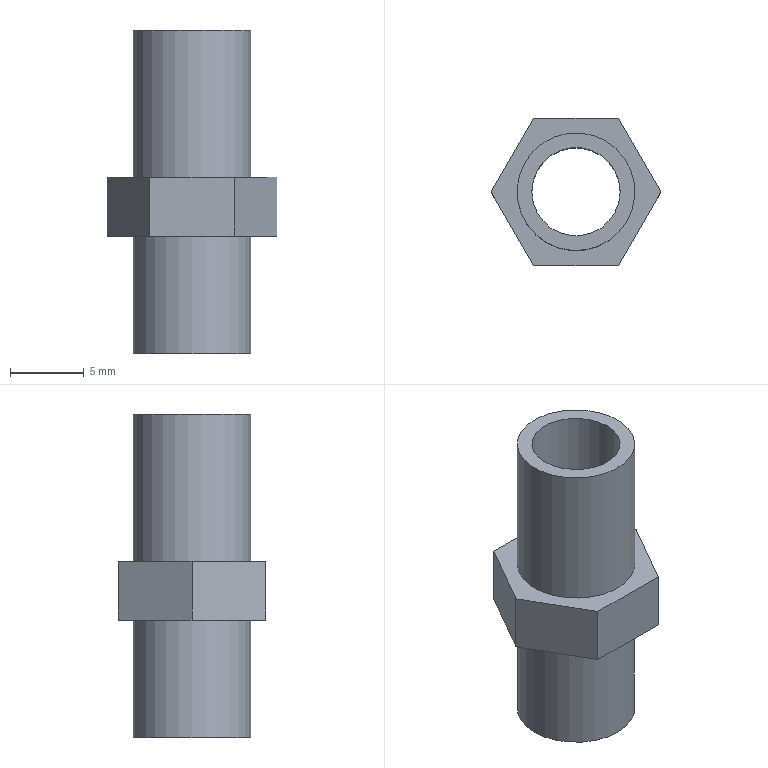Component | NX | PIPE_CAP_2_2 | 1 solid | 13 faces | box 11.55 x 10 x 22 mm | volume 629 mm3 | plane 10 | cylinder 3 | commonest cylinder face diameters 8 x2 6 x1
STEP:
#1=CARTESIAN_POINT('',(0.,0.,0.));
#2=DIRECTION('',(0.,0.,1.));
#3=DIRECTION('',(1.,0.,0.));
#4=AXIS2_PLACEMENT_3D('',#1,#2,#3);
#5=CARTESIAN_POINT('',(-114.5,-59.,24.5));
#6=VERTEX_POINT('',#5);
#7=CARTESIAN_POINT('',(-108.5,-59.,24.5));
#8=VERTEX_POINT('',#7);
#9=CARTESIAN_POINT('',(-111.5,-59.,24.5));
#10=DIRECTION('',(0.,0.,-1.));
#11=DIRECTION('',(-1.,0.,0.));
#12=AXIS2_PLACEMENT_3D('',#9,#10,#11);
#13=CIRCLE('',#12,3.);
#14=CARTESIAN_POINT('',(-111.5,-59.,24.5));
#15=DIRECTION('',(0.,0.,-1.));
#16=DIRECTION('',(-1.,0.,0.));
#17=AXIS2_PLACEMENT_3D('',#14,#15,#16);
#18=PLANE('',#17);
#19=CARTESIAN_POINT('',(0.,0.));
#20=DIRECTION('',(1.,0.));
#21=AXIS2_PLACEMENT_2D('',#19,#20);
#22=CIRCLE('',#21,3.);
#23=(GEOMETRIC_REPRESENTATION_CONTEXT(2)PARAMETRIC_REPRESENTATION_CONTEXT()REPRESENTATION_CONTEXT('',''));
#24=DEFINITIONAL_REPRESENTATION('',(#22),#23);
#25=PCURVE('',#18,#24);
#26=CARTESIAN_POINT('',(-111.5,-59.,-3.5));
#27=DIRECTION('',(0.,0.,1.));
#28=DIRECTION('',(1.,0.,0.));
#29=AXIS2_PLACEMENT_3D('',#26,#27,#28);
#30=CYLINDRICAL_SURFACE('',#29,3.);
#31=CARTESIAN_POINT('',(3.142,28.));
#32=DIRECTION('',(-1.,0.));
#33=VECTOR('',#32,1.);
#34=LINE('',#31,#33);
#35=(GEOMETRIC_REPRESENTATION_CONTEXT(2)PARAMETRIC_REPRESENTATION_CONTEXT()REPRESENTATION_CONTEXT('',''));
#36=DEFINITIONAL_REPRESENTATION('',(#34),#35);
#37=PCURVE('',#30,#36);
#38=SURFACE_CURVE('',#13,(#25,#37),.PCURVE_S1.);
#39=EDGE_CURVE('',#6,#8,#38,.T.);
#40=ORIENTED_EDGE('',*,*,#39,.F.);
#41=CARTESIAN_POINT('',(-111.5,-59.,24.5));
#42=DIRECTION('',(0.,0.,-1.));
#43=DIRECTION('',(-1.,0.,0.));
#44=AXIS2_PLACEMENT_3D('',#41,#42,#43);
#45=CIRCLE('',#44,3.);
#46=CARTESIAN_POINT('',(0.,0.));
#47=DIRECTION('',(1.,0.));
#48=AXIS2_PLACEMENT_2D('',#46,#47);
#49=CIRCLE('',#48,3.);
#50=(GEOMETRIC_REPRESENTATION_CONTEXT(2)PARAMETRIC_REPRESENTATION_CONTEXT()REPRESENTATION_CONTEXT('',''));
#51=DEFINITIONAL_REPRESENTATION('',(#49),#50);
#52=PCURVE('',#18,#51);
#53=CARTESIAN_POINT('',(9.425,28.));
#54=DIRECTION('',(-1.,0.));
#55=VECTOR('',#54,1.);
#56=LINE('',#53,#55);
#57=(GEOMETRIC_REPRESENTATION_CONTEXT(2)PARAMETRIC_REPRESENTATION_CONTEXT()REPRESENTATION_CONTEXT('',''));
#58=DEFINITIONAL_REPRESENTATION('',(#56),#57);
#59=PCURVE('',#30,#58);
#60=SURFACE_CURVE('',#45,(#52,#59),.PCURVE_S1.);
#61=EDGE_CURVE('',#8,#6,#60,.T.);
#62=ORIENTED_EDGE('',*,*,#61,.F.);
#63=EDGE_LOOP('',(#40,#62));
#64=FACE_BOUND('',#63,.T.);
#65=CARTESIAN_POINT('',(-107.5,-59.,24.5));
#66=VERTEX_POINT('',#65);
#67=CARTESIAN_POINT('',(-111.5,-59.,24.5));
#68=DIRECTION('',(0.,0.,1.));
#69=DIRECTION('',(1.,0.,0.));
#70=AXIS2_PLACEMENT_3D('',#67,#68,#69);
#71=CIRCLE('',#70,4.);
#72=CARTESIAN_POINT('',(-4.,0.));
#73=CARTESIAN_POINT('',(-4.,6.928));
#74=CARTESIAN_POINT('',(2.,3.464));
#75=CARTESIAN_POINT('',(8.,0.));
#76=CARTESIAN_POINT('',(2.,-3.464));
#77=CARTESIAN_POINT('',(-4.,-6.928));
#78=CARTESIAN_POINT('',(-4.,0.));
#79=(BOUNDED_CURVE()B_SPLINE_CURVE(2,(#72,#73,#74,#75,#76,#77,#78),.UNSPECIFIED.,.T.,.F.)B_SPLINE_CURVE_WITH_KNOTS((1,2,2,2,2,1),(-2.094,0.,2.094,4.189,6.283,8.378),.UNSPECIFIED.)CURVE()GEOMETRIC_REPRESENTATION_ITEM()RATIONAL_B_SPLINE_CURVE((1.,0.5,1.,0.5,1.,0.5,1.))REPRESENTATION_ITEM(''));
#80=(GEOMETRIC_REPRESENTATION_CONTEXT(2)PARAMETRIC_REPRESENTATION_CONTEXT()REPRESENTATION_CONTEXT('',''));
#81=DEFINITIONAL_REPRESENTATION('',(#79),#80);
#82=PCURVE('',#18,#81);
#83=CARTESIAN_POINT('',(-111.5,-59.,24.5));
#84=DIRECTION('',(0.,0.,1.));
#85=DIRECTION('',(1.,0.,0.));
#86=AXIS2_PLACEMENT_3D('',#83,#84,#85);
#87=CYLINDRICAL_SURFACE('',#86,4.);
#88=CARTESIAN_POINT('',(0.,0.));
#89=DIRECTION('',(1.,0.));
#90=VECTOR('',#89,1.);
#91=LINE('',#88,#90);
#92=(GEOMETRIC_REPRESENTATION_CONTEXT(2)PARAMETRIC_REPRESENTATION_CONTEXT()REPRESENTATION_CONTEXT('',''));
#93=DEFINITIONAL_REPRESENTATION('',(#91),#92);
#94=PCURVE('',#87,#93);
#95=SURFACE_CURVE('',#71,(#82,#94),.PCURVE_S1.);
#96=EDGE_CURVE('',#66,#66,#95,.T.);
#97=ORIENTED_EDGE('',*,*,#96,.F.);
#98=EDGE_LOOP('',(#97));
#99=FACE_BOUND('',#98,.T.);
#100=ADVANCED_FACE('',(#64,#99),#18,.T.);
#101=CARTESIAN_POINT('',(-107.5,-59.,32.5));
#102=VERTEX_POINT('',#101);
#103=CARTESIAN_POINT('',(-111.5,-59.,32.5));
#104=DIRECTION('',(0.,0.,-1.));
#105=DIRECTION('',(1.,0.,0.));
#106=AXIS2_PLACEMENT_3D('',#103,#104,#105);
#107=CIRCLE('',#106,4.);
#108=CARTESIAN_POINT('',(6.283,8.));
#109=DIRECTION('',(-1.,0.));
#110=VECTOR('',#109,1.);
#111=LINE('',#108,#110);
#112=(GEOMETRIC_REPRESENTATION_CONTEXT(2)PARAMETRIC_REPRESENTATION_CONTEXT()REPRESENTATION_CONTEXT('',''));
#113=DEFINITIONAL_REPRESENTATION('',(#111),#112);
#114=PCURVE('',#87,#113);
#115=CARTESIAN_POINT('',(-111.5,-59.,32.5));
#116=DIRECTION('',(0.,0.,-1.));
#117=DIRECTION('',(-1.,0.,0.));
#118=AXIS2_PLACEMENT_3D('',#115,#116,#117);
#119=PLANE('',#118);
#120=CARTESIAN_POINT('',(0.,0.));
#121=DIRECTION('',(-1.,0.));
#122=AXIS2_PLACEMENT_2D('',#120,#121);
#123=CIRCLE('',#122,4.);
#124=(GEOMETRIC_REPRESENTATION_CONTEXT(2)PARAMETRIC_REPRESENTATION_CONTEXT()REPRESENTATION_CONTEXT('',''));
#125=DEFINITIONAL_REPRESENTATION('',(#123),#124);
#126=PCURVE('',#119,#125);
#127=SURFACE_CURVE('',#107,(#114,#126),.PCURVE_S1.);
#128=EDGE_CURVE('',#102,#102,#127,.T.);
#129=ORIENTED_EDGE('',*,*,#128,.T.);
#130=CARTESIAN_POINT('',(-107.5,-59.,24.5));
#131=CARTESIAN_POINT('',(-107.5,-59.,32.5));
#132=B_SPLINE_CURVE_WITH_KNOTS('',1,(#130,#131),.UNSPECIFIED.,.F.,.F.,(2,2),(0.,8.),.PIECEWISE_BEZIER_KNOTS.);
#133=CARTESIAN_POINT('',(0.,0.));
#134=DIRECTION('',(0.,1.));
#135=VECTOR('',#134,1.);
#136=LINE('',#133,#135);
#137=(GEOMETRIC_REPRESENTATION_CONTEXT(2)PARAMETRIC_REPRESENTATION_CONTEXT()REPRESENTATION_CONTEXT('',''));
#138=DEFINITIONAL_REPRESENTATION('',(#136),#137);
#139=PCURVE('',#87,#138);
#140=CARTESIAN_POINT('',(6.283,0.));
#141=DIRECTION('',(0.,1.));
#142=VECTOR('',#141,1.);
#143=LINE('',#140,#142);
#144=(GEOMETRIC_REPRESENTATION_CONTEXT(2)PARAMETRIC_REPRESENTATION_CONTEXT()REPRESENTATION_CONTEXT('',''));
#145=DEFINITIONAL_REPRESENTATION('',(#143),#144);
#146=PCURVE('',#87,#145);
#147=SEAM_CURVE('',#132,(#139,#146),.PCURVE_S1.);
#148=EDGE_CURVE('',#66,#102,#147,.T.);
#149=ORIENTED_EDGE('',*,*,#148,.F.);
#150=ORIENTED_EDGE('',*,*,#96,.T.);
#151=ORIENTED_EDGE('',*,*,#148,.T.);
#152=EDGE_LOOP('',(#129,#149,#150,#151));
#153=FACE_BOUND('',#152,.T.);
#154=ADVANCED_FACE('',(#153),#87,.T.);
#155=CARTESIAN_POINT('',(-108.613,-54.,32.5));
#156=VERTEX_POINT('',#155);
#157=CARTESIAN_POINT('',(-105.726,-59.,32.5));
#158=VERTEX_POINT('',#157);
#159=CARTESIAN_POINT('',(-108.613,-54.,32.5));
#160=DIRECTION('',(0.5,-0.866,0.));
#161=VECTOR('',#160,1.);
#162=LINE('',#159,#161);
#163=CARTESIAN_POINT('',(-108.613,-54.,36.5));
#164=DIRECTION('',(0.866,0.5,0.));
#165=DIRECTION('',(-0.5,0.866,0.));
#166=AXIS2_PLACEMENT_3D('',#163,#164,#165);
#167=PLANE('',#166);
#168=CARTESIAN_POINT('',(0.,-4.));
#169=DIRECTION('',(-1.,0.));
#170=VECTOR('',#169,1.);
#171=LINE('',#168,#170);
#172=(GEOMETRIC_REPRESENTATION_CONTEXT(2)PARAMETRIC_REPRESENTATION_CONTEXT()REPRESENTATION_CONTEXT('',''));
#173=DEFINITIONAL_REPRESENTATION('',(#171),#172);
#174=PCURVE('',#167,#173);
#175=CARTESIAN_POINT('',(-2.887,5.));
#176=DIRECTION('',(-0.5,-0.866));
#177=VECTOR('',#176,1.);
#178=LINE('',#175,#177);
#179=(GEOMETRIC_REPRESENTATION_CONTEXT(2)PARAMETRIC_REPRESENTATION_CONTEXT()REPRESENTATION_CONTEXT('',''));
#180=DEFINITIONAL_REPRESENTATION('',(#178),#179);
#181=PCURVE('',#119,#180);
#182=SURFACE_CURVE('',#162,(#174,#181),.PCURVE_S1.);
#183=EDGE_CURVE('',#156,#158,#182,.T.);
#184=ORIENTED_EDGE('',*,*,#183,.F.);
#185=CARTESIAN_POINT('',(-108.613,-54.,36.5));
#186=VERTEX_POINT('',#185);
#187=CARTESIAN_POINT('',(-108.613,-54.,36.5));
#188=DIRECTION('',(0.,0.,-1.));
#189=VECTOR('',#188,1.);
#190=LINE('',#187,#189);
#191=CARTESIAN_POINT('',(0.,0.));
#192=DIRECTION('',(0.,-1.));
#193=VECTOR('',#192,1.);
#194=LINE('',#191,#193);
#195=(GEOMETRIC_REPRESENTATION_CONTEXT(2)PARAMETRIC_REPRESENTATION_CONTEXT()REPRESENTATION_CONTEXT('',''));
#196=DEFINITIONAL_REPRESENTATION('',(#194),#195);
#197=PCURVE('',#167,#196);
#198=CARTESIAN_POINT('',(-114.387,-54.,36.5));
#199=DIRECTION('',(0.,1.,0.));
#200=DIRECTION('',(0.,0.,1.));
#201=AXIS2_PLACEMENT_3D('',#198,#199,#200);
#202=PLANE('',#201);
#203=CARTESIAN_POINT('',(0.,5.774));
#204=DIRECTION('',(-1.,0.));
#205=VECTOR('',#204,1.);
#206=LINE('',#203,#205);
#207=(GEOMETRIC_REPRESENTATION_CONTEXT(2)PARAMETRIC_REPRESENTATION_CONTEXT()REPRESENTATION_CONTEXT('',''));
#208=DEFINITIONAL_REPRESENTATION('',(#206),#207);
#209=PCURVE('',#202,#208);
#210=SURFACE_CURVE('',#190,(#197,#209),.PCURVE_S1.);
#211=EDGE_CURVE('',#186,#156,#210,.T.);
#212=ORIENTED_EDGE('',*,*,#211,.F.);
#213=CARTESIAN_POINT('',(-105.726,-59.,36.5));
#214=VERTEX_POINT('',#213);
#215=CARTESIAN_POINT('',(-108.613,-54.,36.5));
#216=DIRECTION('',(0.5,-0.866,0.));
#217=VECTOR('',#216,1.);
#218=LINE('',#215,#217);
#219=CARTESIAN_POINT('',(0.,0.));
#220=DIRECTION('',(-1.,0.));
#221=VECTOR('',#220,1.);
#222=LINE('',#219,#221);
#223=(GEOMETRIC_REPRESENTATION_CONTEXT(2)PARAMETRIC_REPRESENTATION_CONTEXT()REPRESENTATION_CONTEXT('',''));
#224=DEFINITIONAL_REPRESENTATION('',(#222),#223);
#225=PCURVE('',#167,#224);
#226=CARTESIAN_POINT('',(-111.5,-59.,36.5));
#227=DIRECTION('',(0.,0.,-1.));
#228=DIRECTION('',(-1.,0.,0.));
#229=AXIS2_PLACEMENT_3D('',#226,#227,#228);
#230=PLANE('',#229);
#231=CARTESIAN_POINT('',(-2.887,5.));
#232=DIRECTION('',(-0.5,-0.866));
#233=VECTOR('',#232,1.);
#234=LINE('',#231,#233);
#235=(GEOMETRIC_REPRESENTATION_CONTEXT(2)PARAMETRIC_REPRESENTATION_CONTEXT()REPRESENTATION_CONTEXT('',''));
#236=DEFINITIONAL_REPRESENTATION('',(#234),#235);
#237=PCURVE('',#230,#236);
#238=SURFACE_CURVE('',#218,(#225,#237),.PCURVE_S1.);
#239=EDGE_CURVE('',#186,#214,#238,.T.);
#240=ORIENTED_EDGE('',*,*,#239,.T.);
#241=CARTESIAN_POINT('',(-105.726,-59.,36.5));
#242=DIRECTION('',(0.,0.,-1.));
#243=VECTOR('',#242,1.);
#244=LINE('',#241,#243);
#245=CARTESIAN_POINT('',(-5.774,0.));
#246=DIRECTION('',(0.,-1.));
#247=VECTOR('',#246,1.);
#248=LINE('',#245,#247);
#249=(GEOMETRIC_REPRESENTATION_CONTEXT(2)PARAMETRIC_REPRESENTATION_CONTEXT()REPRESENTATION_CONTEXT('',''));
#250=DEFINITIONAL_REPRESENTATION('',(#248),#249);
#251=PCURVE('',#167,#250);
#252=CARTESIAN_POINT('',(-105.726,-59.,36.5));
#253=DIRECTION('',(0.866,-0.5,0.));
#254=DIRECTION('',(0.5,0.866,0.));
#255=AXIS2_PLACEMENT_3D('',#252,#253,#254);
#256=PLANE('',#255);
#257=CARTESIAN_POINT('',(0.,0.));
#258=DIRECTION('',(0.,-1.));
#259=VECTOR('',#258,1.);
#260=LINE('',#257,#259);
#261=(GEOMETRIC_REPRESENTATION_CONTEXT(2)PARAMETRIC_REPRESENTATION_CONTEXT()REPRESENTATION_CONTEXT('',''));
#262=DEFINITIONAL_REPRESENTATION('',(#260),#261);
#263=PCURVE('',#256,#262);
#264=SURFACE_CURVE('',#244,(#251,#263),.PCURVE_S1.);
#265=EDGE_CURVE('',#214,#158,#264,.T.);
#266=ORIENTED_EDGE('',*,*,#265,.T.);
#267=EDGE_LOOP('',(#184,#212,#240,#266));
#268=FACE_BOUND('',#267,.T.);
#269=ADVANCED_FACE('',(#268),#167,.T.);
#270=CARTESIAN_POINT('',(-108.613,-64.,32.5));
#271=VERTEX_POINT('',#270);
#272=CARTESIAN_POINT('',(-105.726,-59.,32.5));
#273=DIRECTION('',(-0.5,-0.866,0.));
#274=VECTOR('',#273,1.);
#275=LINE('',#272,#274);
#276=CARTESIAN_POINT('',(0.,-4.));
#277=DIRECTION('',(-1.,0.));
#278=VECTOR('',#277,1.);
#279=LINE('',#276,#278);
#280=(GEOMETRIC_REPRESENTATION_CONTEXT(2)PARAMETRIC_REPRESENTATION_CONTEXT()REPRESENTATION_CONTEXT('',''));
#281=DEFINITIONAL_REPRESENTATION('',(#279),#280);
#282=PCURVE('',#256,#281);
#283=CARTESIAN_POINT('',(-5.774,0.));
#284=DIRECTION('',(0.5,-0.866));
#285=VECTOR('',#284,1.);
#286=LINE('',#283,#285);
#287=(GEOMETRIC_REPRESENTATION_CONTEXT(2)PARAMETRIC_REPRESENTATION_CONTEXT()REPRESENTATION_CONTEXT('',''));
#288=DEFINITIONAL_REPRESENTATION('',(#286),#287);
#289=PCURVE('',#119,#288);
#290=SURFACE_CURVE('',#275,(#282,#289),.PCURVE_S1.);
#291=EDGE_CURVE('',#158,#271,#290,.T.);
#292=ORIENTED_EDGE('',*,*,#291,.F.);
#293=ORIENTED_EDGE('',*,*,#265,.F.);
#294=CARTESIAN_POINT('',(-108.613,-64.,36.5));
#295=VERTEX_POINT('',#294);
#296=CARTESIAN_POINT('',(-105.726,-59.,36.5));
#297=DIRECTION('',(-0.5,-0.866,0.));
#298=VECTOR('',#297,1.);
#299=LINE('',#296,#298);
#300=CARTESIAN_POINT('',(0.,0.));
#301=DIRECTION('',(-1.,0.));
#302=VECTOR('',#301,1.);
#303=LINE('',#300,#302);
#304=(GEOMETRIC_REPRESENTATION_CONTEXT(2)PARAMETRIC_REPRESENTATION_CONTEXT()REPRESENTATION_CONTEXT('',''));
#305=DEFINITIONAL_REPRESENTATION('',(#303),#304);
#306=PCURVE('',#256,#305);
#307=CARTESIAN_POINT('',(-5.774,0.));
#308=DIRECTION('',(0.5,-0.866));
#309=VECTOR('',#308,1.);
#310=LINE('',#307,#309);
#311=(GEOMETRIC_REPRESENTATION_CONTEXT(2)PARAMETRIC_REPRESENTATION_CONTEXT()REPRESENTATION_CONTEXT('',''));
#312=DEFINITIONAL_REPRESENTATION('',(#310),#311);
#313=PCURVE('',#230,#312);
#314=SURFACE_CURVE('',#299,(#306,#313),.PCURVE_S1.);
#315=EDGE_CURVE('',#214,#295,#314,.T.);
#316=ORIENTED_EDGE('',*,*,#315,.T.);
#317=CARTESIAN_POINT('',(-108.613,-64.,36.5));
#318=DIRECTION('',(0.,0.,-1.));
#319=VECTOR('',#318,1.);
#320=LINE('',#317,#319);
#321=CARTESIAN_POINT('',(-5.774,0.));
#322=DIRECTION('',(0.,-1.));
#323=VECTOR('',#322,1.);
#324=LINE('',#321,#323);
#325=(GEOMETRIC_REPRESENTATION_CONTEXT(2)PARAMETRIC_REPRESENTATION_CONTEXT()REPRESENTATION_CONTEXT('',''));
#326=DEFINITIONAL_REPRESENTATION('',(#324),#325);
#327=PCURVE('',#256,#326);
#328=CARTESIAN_POINT('',(-108.613,-64.,36.5));
#329=DIRECTION('',(-0.,-1.,0.));
#330=DIRECTION('',(1.,-0.,0.));
#331=AXIS2_PLACEMENT_3D('',#328,#329,#330);
#332=PLANE('',#331);
#333=CARTESIAN_POINT('',(0.,0.));
#334=DIRECTION('',(0.,-1.));
#335=VECTOR('',#334,1.);
#336=LINE('',#333,#335);
#337=(GEOMETRIC_REPRESENTATION_CONTEXT(2)PARAMETRIC_REPRESENTATION_CONTEXT()REPRESENTATION_CONTEXT('',''));
#338=DEFINITIONAL_REPRESENTATION('',(#336),#337);
#339=PCURVE('',#332,#338);
#340=SURFACE_CURVE('',#320,(#327,#339),.PCURVE_S1.);
#341=EDGE_CURVE('',#295,#271,#340,.T.);
#342=ORIENTED_EDGE('',*,*,#341,.T.);
#343=EDGE_LOOP('',(#292,#293,#316,#342));
#344=FACE_BOUND('',#343,.T.);
#345=ADVANCED_FACE('',(#344),#256,.T.);
#346=CARTESIAN_POINT('',(-114.387,-64.,32.5));
#347=VERTEX_POINT('',#346);
#348=CARTESIAN_POINT('',(-108.613,-64.,32.5));
#349=DIRECTION('',(-1.,0.,0.));
#350=VECTOR('',#349,1.);
#351=LINE('',#348,#350);
#352=CARTESIAN_POINT('',(0.,-4.));
#353=DIRECTION('',(-1.,0.));
#354=VECTOR('',#353,1.);
#355=LINE('',#352,#354);
#356=(GEOMETRIC_REPRESENTATION_CONTEXT(2)PARAMETRIC_REPRESENTATION_CONTEXT()REPRESENTATION_CONTEXT('',''));
#357=DEFINITIONAL_REPRESENTATION('',(#355),#356);
#358=PCURVE('',#332,#357);
#359=CARTESIAN_POINT('',(-2.887,-5.));
#360=DIRECTION('',(1.,0.));
#361=VECTOR('',#360,1.);
#362=LINE('',#359,#361);
#363=(GEOMETRIC_REPRESENTATION_CONTEXT(2)PARAMETRIC_REPRESENTATION_CONTEXT()REPRESENTATION_CONTEXT('',''));
#364=DEFINITIONAL_REPRESENTATION('',(#362),#363);
#365=PCURVE('',#119,#364);
#366=SURFACE_CURVE('',#351,(#358,#365),.PCURVE_S1.);
#367=EDGE_CURVE('',#271,#347,#366,.T.);
#368=ORIENTED_EDGE('',*,*,#367,.F.);
#369=ORIENTED_EDGE('',*,*,#341,.F.);
#370=CARTESIAN_POINT('',(-114.387,-64.,36.5));
#371=VERTEX_POINT('',#370);
#372=CARTESIAN_POINT('',(-108.613,-64.,36.5));
#373=DIRECTION('',(-1.,0.,0.));
#374=VECTOR('',#373,1.);
#375=LINE('',#372,#374);
#376=CARTESIAN_POINT('',(0.,0.));
#377=DIRECTION('',(-1.,0.));
#378=VECTOR('',#377,1.);
#379=LINE('',#376,#378);
#380=(GEOMETRIC_REPRESENTATION_CONTEXT(2)PARAMETRIC_REPRESENTATION_CONTEXT()REPRESENTATION_CONTEXT('',''));
#381=DEFINITIONAL_REPRESENTATION('',(#379),#380);
#382=PCURVE('',#332,#381);
#383=CARTESIAN_POINT('',(-2.887,-5.));
#384=DIRECTION('',(1.,0.));
#385=VECTOR('',#384,1.);
#386=LINE('',#383,#385);
#387=(GEOMETRIC_REPRESENTATION_CONTEXT(2)PARAMETRIC_REPRESENTATION_CONTEXT()REPRESENTATION_CONTEXT('',''));
#388=DEFINITIONAL_REPRESENTATION('',(#386),#387);
#389=PCURVE('',#230,#388);
#390=SURFACE_CURVE('',#375,(#382,#389),.PCURVE_S1.);
#391=EDGE_CURVE('',#295,#371,#390,.T.);
#392=ORIENTED_EDGE('',*,*,#391,.T.);
#393=CARTESIAN_POINT('',(-114.387,-64.,36.5));
#394=DIRECTION('',(0.,0.,-1.));
#395=VECTOR('',#394,1.);
#396=LINE('',#393,#395);
#397=CARTESIAN_POINT('',(-5.774,0.));
#398=DIRECTION('',(0.,-1.));
#399=VECTOR('',#398,1.);
#400=LINE('',#397,#399);
#401=(GEOMETRIC_REPRESENTATION_CONTEXT(2)PARAMETRIC_REPRESENTATION_CONTEXT()REPRESENTATION_CONTEXT('',''));
#402=DEFINITIONAL_REPRESENTATION('',(#400),#401);
#403=PCURVE('',#332,#402);
#404=CARTESIAN_POINT('',(-114.387,-64.,36.5));
#405=DIRECTION('',(-0.866,-0.5,0.));
#406=DIRECTION('',(0.5,-0.866,0.));
#407=AXIS2_PLACEMENT_3D('',#404,#405,#406);
#408=PLANE('',#407);
#409=CARTESIAN_POINT('',(0.,0.));
#410=DIRECTION('',(0.,-1.));
#411=VECTOR('',#410,1.);
#412=LINE('',#409,#411);
#413=(GEOMETRIC_REPRESENTATION_CONTEXT(2)PARAMETRIC_REPRESENTATION_CONTEXT()REPRESENTATION_CONTEXT('',''));
#414=DEFINITIONAL_REPRESENTATION('',(#412),#413);
#415=PCURVE('',#408,#414);
#416=SURFACE_CURVE('',#396,(#403,#415),.PCURVE_S1.);
#417=EDGE_CURVE('',#371,#347,#416,.T.);
#418=ORIENTED_EDGE('',*,*,#417,.T.);
#419=EDGE_LOOP('',(#368,#369,#392,#418));
#420=FACE_BOUND('',#419,.T.);
#421=ADVANCED_FACE('',(#420),#332,.T.);
#422=CARTESIAN_POINT('',(-117.274,-59.,32.5));
#423=VERTEX_POINT('',#422);
#424=CARTESIAN_POINT('',(-114.387,-64.,32.5));
#425=DIRECTION('',(-0.5,0.866,0.));
#426=VECTOR('',#425,1.);
#427=LINE('',#424,#426);
#428=CARTESIAN_POINT('',(0.,-4.));
#429=DIRECTION('',(-1.,0.));
#430=VECTOR('',#429,1.);
#431=LINE('',#428,#430);
#432=(GEOMETRIC_REPRESENTATION_CONTEXT(2)PARAMETRIC_REPRESENTATION_CONTEXT()REPRESENTATION_CONTEXT('',''));
#433=DEFINITIONAL_REPRESENTATION('',(#431),#432);
#434=PCURVE('',#408,#433);
#435=CARTESIAN_POINT('',(2.887,-5.));
#436=DIRECTION('',(0.5,0.866));
#437=VECTOR('',#436,1.);
#438=LINE('',#435,#437);
#439=(GEOMETRIC_REPRESENTATION_CONTEXT(2)PARAMETRIC_REPRESENTATION_CONTEXT()REPRESENTATION_CONTEXT('',''));
#440=DEFINITIONAL_REPRESENTATION('',(#438),#439);
#441=PCURVE('',#119,#440);
#442=SURFACE_CURVE('',#427,(#434,#441),.PCURVE_S1.);
#443=EDGE_CURVE('',#347,#423,#442,.T.);
#444=ORIENTED_EDGE('',*,*,#443,.F.);
#445=ORIENTED_EDGE('',*,*,#417,.F.);
#446=CARTESIAN_POINT('',(-117.274,-59.,36.5));
#447=VERTEX_POINT('',#446);
#448=CARTESIAN_POINT('',(-114.387,-64.,36.5));
#449=DIRECTION('',(-0.5,0.866,0.));
#450=VECTOR('',#449,1.);
#451=LINE('',#448,#450);
#452=CARTESIAN_POINT('',(0.,0.));
#453=DIRECTION('',(-1.,0.));
#454=VECTOR('',#453,1.);
#455=LINE('',#452,#454);
#456=(GEOMETRIC_REPRESENTATION_CONTEXT(2)PARAMETRIC_REPRESENTATION_CONTEXT()REPRESENTATION_CONTEXT('',''));
#457=DEFINITIONAL_REPRESENTATION('',(#455),#456);
#458=PCURVE('',#408,#457);
#459=CARTESIAN_POINT('',(2.887,-5.));
#460=DIRECTION('',(0.5,0.866));
#461=VECTOR('',#460,1.);
#462=LINE('',#459,#461);
#463=(GEOMETRIC_REPRESENTATION_CONTEXT(2)PARAMETRIC_REPRESENTATION_CONTEXT()REPRESENTATION_CONTEXT('',''));
#464=DEFINITIONAL_REPRESENTATION('',(#462),#463);
#465=PCURVE('',#230,#464);
#466=SURFACE_CURVE('',#451,(#458,#465),.PCURVE_S1.);
#467=EDGE_CURVE('',#371,#447,#466,.T.);
#468=ORIENTED_EDGE('',*,*,#467,.T.);
#469=CARTESIAN_POINT('',(-117.274,-59.,36.5));
#470=DIRECTION('',(0.,0.,-1.));
#471=VECTOR('',#470,1.);
#472=LINE('',#469,#471);
#473=CARTESIAN_POINT('',(-5.774,0.));
#474=DIRECTION('',(0.,-1.));
#475=VECTOR('',#474,1.);
#476=LINE('',#473,#475);
#477=(GEOMETRIC_REPRESENTATION_CONTEXT(2)PARAMETRIC_REPRESENTATION_CONTEXT()REPRESENTATION_CONTEXT('',''));
#478=DEFINITIONAL_REPRESENTATION('',(#476),#477);
#479=PCURVE('',#408,#478);
#480=CARTESIAN_POINT('',(-117.274,-59.,36.5));
#481=DIRECTION('',(-0.866,0.5,0.));
#482=DIRECTION('',(-0.5,-0.866,0.));
#483=AXIS2_PLACEMENT_3D('',#480,#481,#482);
#484=PLANE('',#483);
#485=CARTESIAN_POINT('',(0.,0.));
#486=DIRECTION('',(0.,-1.));
#487=VECTOR('',#486,1.);
#488=LINE('',#485,#487);
#489=(GEOMETRIC_REPRESENTATION_CONTEXT(2)PARAMETRIC_REPRESENTATION_CONTEXT()REPRESENTATION_CONTEXT('',''));
#490=DEFINITIONAL_REPRESENTATION('',(#488),#489);
#491=PCURVE('',#484,#490);
#492=SURFACE_CURVE('',#472,(#479,#491),.PCURVE_S1.);
#493=EDGE_CURVE('',#447,#423,#492,.T.);
#494=ORIENTED_EDGE('',*,*,#493,.T.);
#495=EDGE_LOOP('',(#444,#445,#468,#494));
#496=FACE_BOUND('',#495,.T.);
#497=ADVANCED_FACE('',(#496),#408,.T.);
#498=CARTESIAN_POINT('',(-114.387,-54.,32.5));
#499=VERTEX_POINT('',#498);
#500=CARTESIAN_POINT('',(-117.274,-59.,32.5));
#501=DIRECTION('',(0.5,0.866,0.));
#502=VECTOR('',#501,1.);
#503=LINE('',#500,#502);
#504=CARTESIAN_POINT('',(0.,-4.));
#505=DIRECTION('',(-1.,0.));
#506=VECTOR('',#505,1.);
#507=LINE('',#504,#506);
#508=(GEOMETRIC_REPRESENTATION_CONTEXT(2)PARAMETRIC_REPRESENTATION_CONTEXT()REPRESENTATION_CONTEXT('',''));
#509=DEFINITIONAL_REPRESENTATION('',(#507),#508);
#510=PCURVE('',#484,#509);
#511=CARTESIAN_POINT('',(5.774,0.));
#512=DIRECTION('',(-0.5,0.866));
#513=VECTOR('',#512,1.);
#514=LINE('',#511,#513);
#515=(GEOMETRIC_REPRESENTATION_CONTEXT(2)PARAMETRIC_REPRESENTATION_CONTEXT()REPRESENTATION_CONTEXT('',''));
#516=DEFINITIONAL_REPRESENTATION('',(#514),#515);
#517=PCURVE('',#119,#516);
#518=SURFACE_CURVE('',#503,(#510,#517),.PCURVE_S1.);
#519=EDGE_CURVE('',#423,#499,#518,.T.);
#520=ORIENTED_EDGE('',*,*,#519,.F.);
#521=ORIENTED_EDGE('',*,*,#493,.F.);
#522=CARTESIAN_POINT('',(-114.387,-54.,36.5));
#523=VERTEX_POINT('',#522);
#524=CARTESIAN_POINT('',(-117.274,-59.,36.5));
#525=DIRECTION('',(0.5,0.866,0.));
#526=VECTOR('',#525,1.);
#527=LINE('',#524,#526);
#528=CARTESIAN_POINT('',(0.,0.));
#529=DIRECTION('',(-1.,0.));
#530=VECTOR('',#529,1.);
#531=LINE('',#528,#530);
#532=(GEOMETRIC_REPRESENTATION_CONTEXT(2)PARAMETRIC_REPRESENTATION_CONTEXT()REPRESENTATION_CONTEXT('',''));
#533=DEFINITIONAL_REPRESENTATION('',(#531),#532);
#534=PCURVE('',#484,#533);
#535=CARTESIAN_POINT('',(5.774,0.));
#536=DIRECTION('',(-0.5,0.866));
#537=VECTOR('',#536,1.);
#538=LINE('',#535,#537);
#539=(GEOMETRIC_REPRESENTATION_CONTEXT(2)PARAMETRIC_REPRESENTATION_CONTEXT()REPRESENTATION_CONTEXT('',''));
#540=DEFINITIONAL_REPRESENTATION('',(#538),#539);
#541=PCURVE('',#230,#540);
#542=SURFACE_CURVE('',#527,(#534,#541),.PCURVE_S1.);
#543=EDGE_CURVE('',#447,#523,#542,.T.);
#544=ORIENTED_EDGE('',*,*,#543,.T.);
#545=CARTESIAN_POINT('',(-114.387,-54.,36.5));
#546=DIRECTION('',(0.,0.,-1.));
#547=VECTOR('',#546,1.);
#548=LINE('',#545,#547);
#549=CARTESIAN_POINT('',(-5.774,0.));
#550=DIRECTION('',(0.,-1.));
#551=VECTOR('',#550,1.);
#552=LINE('',#549,#551);
#553=(GEOMETRIC_REPRESENTATION_CONTEXT(2)PARAMETRIC_REPRESENTATION_CONTEXT()REPRESENTATION_CONTEXT('',''));
#554=DEFINITIONAL_REPRESENTATION('',(#552),#553);
#555=PCURVE('',#484,#554);
#556=CARTESIAN_POINT('',(0.,0.));
#557=DIRECTION('',(-1.,0.));
#558=VECTOR('',#557,1.);
#559=LINE('',#556,#558);
#560=(GEOMETRIC_REPRESENTATION_CONTEXT(2)PARAMETRIC_REPRESENTATION_CONTEXT()REPRESENTATION_CONTEXT('',''));
#561=DEFINITIONAL_REPRESENTATION('',(#559),#560);
#562=PCURVE('',#202,#561);
#563=SURFACE_CURVE('',#548,(#555,#562),.PCURVE_S1.);
#564=EDGE_CURVE('',#523,#499,#563,.T.);
#565=ORIENTED_EDGE('',*,*,#564,.T.);
#566=EDGE_LOOP('',(#520,#521,#544,#565));
#567=FACE_BOUND('',#566,.T.);
#568=ADVANCED_FACE('',(#567),#484,.T.);
#569=CARTESIAN_POINT('',(-114.387,-54.,32.5));
#570=DIRECTION('',(1.,0.,0.));
#571=VECTOR('',#570,1.);
#572=LINE('',#569,#571);
#573=CARTESIAN_POINT('',(-4.,0.));
#574=DIRECTION('',(0.,1.));
#575=VECTOR('',#574,1.);
#576=LINE('',#573,#575);
#577=(GEOMETRIC_REPRESENTATION_CONTEXT(2)PARAMETRIC_REPRESENTATION_CONTEXT()REPRESENTATION_CONTEXT('',''));
#578=DEFINITIONAL_REPRESENTATION('',(#576),#577);
#579=PCURVE('',#202,#578);
#580=CARTESIAN_POINT('',(2.887,5.));
#581=DIRECTION('',(-1.,0.));
#582=VECTOR('',#581,1.);
#583=LINE('',#580,#582);
#584=(GEOMETRIC_REPRESENTATION_CONTEXT(2)PARAMETRIC_REPRESENTATION_CONTEXT()REPRESENTATION_CONTEXT('',''));
#585=DEFINITIONAL_REPRESENTATION('',(#583),#584);
#586=PCURVE('',#119,#585);
#587=SURFACE_CURVE('',#572,(#579,#586),.PCURVE_S1.);
#588=EDGE_CURVE('',#499,#156,#587,.T.);
#589=ORIENTED_EDGE('',*,*,#588,.F.);
#590=ORIENTED_EDGE('',*,*,#564,.F.);
#591=CARTESIAN_POINT('',(-114.387,-54.,36.5));
#592=DIRECTION('',(1.,0.,0.));
#593=VECTOR('',#592,1.);
#594=LINE('',#591,#593);
#595=CARTESIAN_POINT('',(0.,0.));
#596=DIRECTION('',(0.,1.));
#597=VECTOR('',#596,1.);
#598=LINE('',#595,#597);
#599=(GEOMETRIC_REPRESENTATION_CONTEXT(2)PARAMETRIC_REPRESENTATION_CONTEXT()REPRESENTATION_CONTEXT('',''));
#600=DEFINITIONAL_REPRESENTATION('',(#598),#599);
#601=PCURVE('',#202,#600);
#602=CARTESIAN_POINT('',(2.887,5.));
#603=DIRECTION('',(-1.,0.));
#604=VECTOR('',#603,1.);
#605=LINE('',#602,#604);
#606=(GEOMETRIC_REPRESENTATION_CONTEXT(2)PARAMETRIC_REPRESENTATION_CONTEXT()REPRESENTATION_CONTEXT('',''));
#607=DEFINITIONAL_REPRESENTATION('',(#605),#606);
#608=PCURVE('',#230,#607);
#609=SURFACE_CURVE('',#594,(#601,#608),.PCURVE_S1.);
#610=EDGE_CURVE('',#523,#186,#609,.T.);
#611=ORIENTED_EDGE('',*,*,#610,.T.);
#612=ORIENTED_EDGE('',*,*,#211,.T.);
#613=EDGE_LOOP('',(#589,#590,#611,#612));
#614=FACE_BOUND('',#613,.T.);
#615=ADVANCED_FACE('',(#614),#202,.T.);
#616=CARTESIAN_POINT('',(-109.5,-55.536,36.5));
#617=VERTEX_POINT('',#616);
#618=CARTESIAN_POINT('',(-111.5,-59.,36.5));
#619=DIRECTION('',(0.,0.,-1.));
#620=DIRECTION('',(0.5,0.866,0.));
#621=AXIS2_PLACEMENT_3D('',#618,#619,#620);
#622=CIRCLE('',#621,4.);
#623=CARTESIAN_POINT('',(0.,0.));
#624=DIRECTION('',(-0.5,0.866));
#625=AXIS2_PLACEMENT_2D('',#623,#624);
#626=CIRCLE('',#625,4.);
#627=(GEOMETRIC_REPRESENTATION_CONTEXT(2)PARAMETRIC_REPRESENTATION_CONTEXT()REPRESENTATION_CONTEXT('',''));
#628=DEFINITIONAL_REPRESENTATION('',(#626),#627);
#629=PCURVE('',#230,#628);
#630=CARTESIAN_POINT('',(-111.5,-59.,46.5));
#631=DIRECTION('',(0.,0.,-1.));
#632=DIRECTION('',(-1.,0.,0.));
#633=AXIS2_PLACEMENT_3D('',#630,#631,#632);
#634=CYLINDRICAL_SURFACE('',#633,4.);
#635=CARTESIAN_POINT('',(2.094,10.));
#636=DIRECTION('',(1.,0.));
#637=VECTOR('',#636,1.);
#638=LINE('',#635,#637);
#639=(GEOMETRIC_REPRESENTATION_CONTEXT(2)PARAMETRIC_REPRESENTATION_CONTEXT()REPRESENTATION_CONTEXT('',''));
#640=DEFINITIONAL_REPRESENTATION('',(#638),#639);
#641=PCURVE('',#634,#640);
#642=SURFACE_CURVE('',#622,(#629,#641),.PCURVE_S1.);
#643=EDGE_CURVE('',#617,#617,#642,.T.);
#644=ORIENTED_EDGE('',*,*,#643,.T.);
#645=EDGE_LOOP('',(#644));
#646=FACE_BOUND('',#645,.T.);
#647=ORIENTED_EDGE('',*,*,#239,.F.);
#648=ORIENTED_EDGE('',*,*,#610,.F.);
#649=ORIENTED_EDGE('',*,*,#543,.F.);
#650=ORIENTED_EDGE('',*,*,#467,.F.);
#651=ORIENTED_EDGE('',*,*,#391,.F.);
#652=ORIENTED_EDGE('',*,*,#315,.F.);
#653=EDGE_LOOP('',(#647,#648,#649,#650,#651,#652));
#654=FACE_BOUND('',#653,.T.);
#655=ADVANCED_FACE('',(#646,#654),#230,.F.);
#656=ORIENTED_EDGE('',*,*,#128,.F.);
#657=EDGE_LOOP('',(#656));
#658=FACE_BOUND('',#657,.T.);
#659=ORIENTED_EDGE('',*,*,#183,.T.);
#660=ORIENTED_EDGE('',*,*,#291,.T.);
#661=ORIENTED_EDGE('',*,*,#367,.T.);
#662=ORIENTED_EDGE('',*,*,#443,.T.);
#663=ORIENTED_EDGE('',*,*,#519,.T.);
#664=ORIENTED_EDGE('',*,*,#588,.T.);
#665=EDGE_LOOP('',(#659,#660,#661,#662,#663,#664));
#666=FACE_BOUND('',#665,.T.);
#667=ADVANCED_FACE('',(#658,#666),#119,.T.);
#668=CARTESIAN_POINT('',(-109.5,-55.536,46.5));
#669=VERTEX_POINT('',#668);
#670=CARTESIAN_POINT('',(-111.5,-59.,46.5));
#671=DIRECTION('',(0.,0.,-1.));
#672=DIRECTION('',(0.5,0.866,0.));
#673=AXIS2_PLACEMENT_3D('',#670,#671,#672);
#674=CIRCLE('',#673,4.);
#675=CARTESIAN_POINT('',(2.094,0.));
#676=DIRECTION('',(1.,0.));
#677=VECTOR('',#676,1.);
#678=LINE('',#675,#677);
#679=(GEOMETRIC_REPRESENTATION_CONTEXT(2)PARAMETRIC_REPRESENTATION_CONTEXT()REPRESENTATION_CONTEXT('',''));
#680=DEFINITIONAL_REPRESENTATION('',(#678),#679);
#681=PCURVE('',#634,#680);
#682=CARTESIAN_POINT('',(-111.5,-59.,46.5));
#683=DIRECTION('',(0.,0.,-1.));
#684=DIRECTION('',(-1.,0.,0.));
#685=AXIS2_PLACEMENT_3D('',#682,#683,#684);
#686=PLANE('',#685);
#687=CARTESIAN_POINT('',(0.,0.));
#688=DIRECTION('',(-0.5,0.866));
#689=AXIS2_PLACEMENT_2D('',#687,#688);
#690=CIRCLE('',#689,4.);
#691=(GEOMETRIC_REPRESENTATION_CONTEXT(2)PARAMETRIC_REPRESENTATION_CONTEXT()REPRESENTATION_CONTEXT('',''));
#692=DEFINITIONAL_REPRESENTATION('',(#690),#691);
#693=PCURVE('',#686,#692);
#694=SURFACE_CURVE('',#674,(#681,#693),.PCURVE_S1.);
#695=EDGE_CURVE('',#669,#669,#694,.T.);
#696=ORIENTED_EDGE('',*,*,#695,.T.);
#697=CARTESIAN_POINT('',(-109.5,-55.536,46.5));
#698=CARTESIAN_POINT('',(-109.5,-55.536,36.5));
#699=B_SPLINE_CURVE_WITH_KNOTS('',1,(#697,#698),.UNSPECIFIED.,.F.,.F.,(2,2),(0.,10.),.PIECEWISE_BEZIER_KNOTS.);
#700=CARTESIAN_POINT('',(8.378,0.));
#701=DIRECTION('',(0.,1.));
#702=VECTOR('',#701,1.);
#703=LINE('',#700,#702);
#704=(GEOMETRIC_REPRESENTATION_CONTEXT(2)PARAMETRIC_REPRESENTATION_CONTEXT()REPRESENTATION_CONTEXT('',''));
#705=DEFINITIONAL_REPRESENTATION('',(#703),#704);
#706=PCURVE('',#634,#705);
#707=CARTESIAN_POINT('',(2.094,0.));
#708=DIRECTION('',(0.,1.));
#709=VECTOR('',#708,1.);
#710=LINE('',#707,#709);
#711=(GEOMETRIC_REPRESENTATION_CONTEXT(2)PARAMETRIC_REPRESENTATION_CONTEXT()REPRESENTATION_CONTEXT('',''));
#712=DEFINITIONAL_REPRESENTATION('',(#710),#711);
#713=PCURVE('',#634,#712);
#714=SEAM_CURVE('',#699,(#706,#713),.PCURVE_S1.);
#715=EDGE_CURVE('',#669,#617,#714,.T.);
#716=ORIENTED_EDGE('',*,*,#715,.T.);
#717=ORIENTED_EDGE('',*,*,#643,.F.);
#718=ORIENTED_EDGE('',*,*,#715,.F.);
#719=EDGE_LOOP('',(#696,#716,#717,#718));
#720=FACE_BOUND('',#719,.T.);
#721=ADVANCED_FACE('',(#720),#634,.T.);
#722=CARTESIAN_POINT('',(-108.5,-59.,46.5));
#723=VERTEX_POINT('',#722);
#724=CARTESIAN_POINT('',(-111.5,-59.,46.5));
#725=DIRECTION('',(0.,0.,1.));
#726=DIRECTION('',(1.,0.,0.));
#727=AXIS2_PLACEMENT_3D('',#724,#725,#726);
#728=CIRCLE('',#727,3.);
#729=CARTESIAN_POINT('',(-3.,0.));
#730=CARTESIAN_POINT('',(-3.,5.196));
#731=CARTESIAN_POINT('',(1.5,2.598));
#732=CARTESIAN_POINT('',(6.,0.));
#733=CARTESIAN_POINT('',(1.5,-2.598));
#734=CARTESIAN_POINT('',(-3.,-5.196));
#735=CARTESIAN_POINT('',(-3.,0.));
#736=(BOUNDED_CURVE()B_SPLINE_CURVE(2,(#729,#730,#731,#732,#733,#734,#735),.UNSPECIFIED.,.T.,.F.)B_SPLINE_CURVE_WITH_KNOTS((1,2,2,2,2,1),(-2.094,0.,2.094,4.189,6.283,8.378),.UNSPECIFIED.)CURVE()GEOMETRIC_REPRESENTATION_ITEM()RATIONAL_B_SPLINE_CURVE((1.,0.5,1.,0.5,1.,0.5,1.))REPRESENTATION_ITEM(''));
#737=(GEOMETRIC_REPRESENTATION_CONTEXT(2)PARAMETRIC_REPRESENTATION_CONTEXT()REPRESENTATION_CONTEXT('',''));
#738=DEFINITIONAL_REPRESENTATION('',(#736),#737);
#739=PCURVE('',#686,#738);
#740=CARTESIAN_POINT('',(0.,50.));
#741=DIRECTION('',(1.,0.));
#742=VECTOR('',#741,1.);
#743=LINE('',#740,#742);
#744=(GEOMETRIC_REPRESENTATION_CONTEXT(2)PARAMETRIC_REPRESENTATION_CONTEXT()REPRESENTATION_CONTEXT('',''));
#745=DEFINITIONAL_REPRESENTATION('',(#743),#744);
#746=PCURVE('',#30,#745);
#747=SURFACE_CURVE('',#728,(#739,#746),.PCURVE_S1.);
#748=EDGE_CURVE('',#723,#723,#747,.T.);
#749=ORIENTED_EDGE('',*,*,#748,.F.);
#750=EDGE_LOOP('',(#749));
#751=FACE_BOUND('',#750,.T.);
#752=ORIENTED_EDGE('',*,*,#695,.F.);
#753=EDGE_LOOP('',(#752));
#754=FACE_BOUND('',#753,.T.);
#755=ADVANCED_FACE('',(#751,#754),#686,.F.);
#756=ORIENTED_EDGE('',*,*,#61,.F.);
#757=CARTESIAN_POINT('',(-108.5,-59.,24.5));
#758=CARTESIAN_POINT('',(-108.5,-59.,46.5));
#759=B_SPLINE_CURVE_WITH_KNOTS('',1,(#757,#758),.UNSPECIFIED.,.F.,.F.,(2,2),(28.,50.),.PIECEWISE_BEZIER_KNOTS.);
#760=CARTESIAN_POINT('',(6.283,0.));
#761=DIRECTION('',(0.,1.));
#762=VECTOR('',#761,1.);
#763=LINE('',#760,#762);
#764=(GEOMETRIC_REPRESENTATION_CONTEXT(2)PARAMETRIC_REPRESENTATION_CONTEXT()REPRESENTATION_CONTEXT('',''));
#765=DEFINITIONAL_REPRESENTATION('',(#763),#764);
#766=PCURVE('',#30,#765);
#767=CARTESIAN_POINT('',(0.,0.));
#768=DIRECTION('',(0.,1.));
#769=VECTOR('',#768,1.);
#770=LINE('',#767,#769);
#771=(GEOMETRIC_REPRESENTATION_CONTEXT(2)PARAMETRIC_REPRESENTATION_CONTEXT()REPRESENTATION_CONTEXT('',''));
#772=DEFINITIONAL_REPRESENTATION('',(#770),#771);
#773=PCURVE('',#30,#772);
#774=SEAM_CURVE('',#759,(#766,#773),.PCURVE_S1.);
#775=EDGE_CURVE('',#8,#723,#774,.T.);
#776=ORIENTED_EDGE('',*,*,#775,.T.);
#777=ORIENTED_EDGE('',*,*,#748,.F.);
#778=ORIENTED_EDGE('',*,*,#775,.F.);
#779=ORIENTED_EDGE('',*,*,#39,.F.);
#780=EDGE_LOOP('',(#756,#776,#777,#778,#779));
#781=FACE_BOUND('',#780,.F.);
#782=ADVANCED_FACE('',(#781),#30,.F.);
#783=CLOSED_SHELL('',(#100,#154,#269,#345,#421,#497,#568,#615,#655,#667,#721,#755,#782));
#784=MANIFOLD_SOLID_BREP('',#783);
#785=(LENGTH_UNIT()NAMED_UNIT(*)SI_UNIT(.MILLI.,.METRE.));
#786=UNCERTAINTY_MEASURE_WITH_UNIT(LENGTH_MEASURE(0.000002),#785,'','');
#787=(NAMED_UNIT(*)PLANE_ANGLE_UNIT()SI_UNIT($,.RADIAN.));
#788=(NAMED_UNIT(*)SI_UNIT($,.STERADIAN.)SOLID_ANGLE_UNIT());
#789=(GEOMETRIC_REPRESENTATION_CONTEXT(3)GLOBAL_UNCERTAINTY_ASSIGNED_CONTEXT((#786))GLOBAL_UNIT_ASSIGNED_CONTEXT((#785,#787,#788))REPRESENTATION_CONTEXT('',''));
#790=ADVANCED_BREP_SHAPE_REPRESENTATION('',(#4,#784),#789);